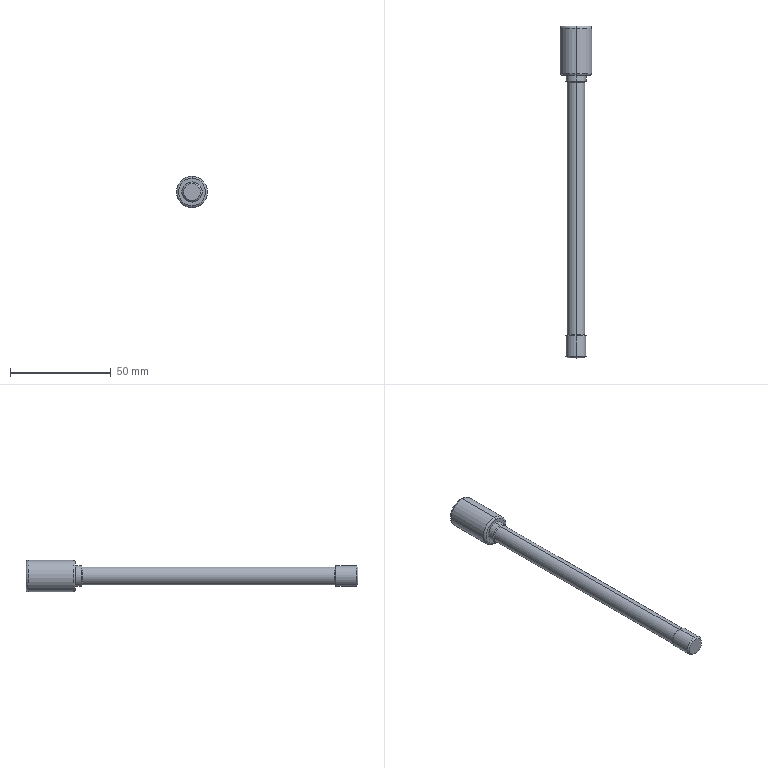Component | SolidWorks | AirTACCylinderFSC_80x75_S_FB-1_FSC80_753-1 | 1 solid | 38 faces | box 15.5 x 164.5 x 15.5 mm | volume 12478 mm3 | plane 16 | cylinder 10 | cone 8 | torus 4 | commonest cylinder face diameters 10 x4 8.9 x2 15.5 x2 8.376 x2
build123d program:
from build123d import *

# Parameters (mm, degrees)
CUT_EXTRUDE1_DEPTH = 4.5


with BuildPart() as part:
    # Sketch1 → Revolve1 (revolve)
    with BuildSketch(Plane.XY, mode=Mode.PRIVATE) as revolve1_sk:
        with BuildLine():
            Line((-24.5, 0), (-24.5, 6.75))
            ThreePointArc((-24.5, 6.75), (-24.207, 7.457), (-23.5, 7.75))
            Line((-23.5, 7.75), (-1, 7.75))
            ThreePointArc((-1, 7.75), (-0.2929, 7.457), (0, 6.75))
            Line((0, 6.75), (0, 0))
            Line((0, 0), (-24.5, 0))
        make_face()
    revolve(revolve1_sk.sketch.rotate(Axis((0, 0, 0), (-1, 0, 0)), 270), axis=Axis((0, 0, 0), (-1, 0, 0)))

    # Sketch2 → Cut-Extrude1 (cut)
    with BuildSketch(Plane(origin=(-24.5, 0, 0), x_dir=(0, 0, -1), z_dir=(1, 0, 0))):
        Polygon((-5, 2.887), (-5, -2.887), (0, -5.774), (5, -2.887), (5, 2.887), (0, 5.774), align=None)
    extrude(amount=CUT_EXTRUDE1_DEPTH, mode=Mode.SUBTRACT)

    # Sketch3 → Cut-Revolve1 (revolve, cut)
    with BuildSketch(Plane.XY, mode=Mode.PRIVATE) as cut_revolve1_sk:
        Polygon((-20, 0), (-20, 5), (-19.188, 4.188), (-0.812, 4.188), (0, 5), (0, 0), align=None)
    revolve(cut_revolve1_sk.sketch.rotate(Axis((0, 0, 0), (-1, 0, 0)), 270), axis=Axis((0, 0, 0), (-1, 0, 0)), mode=Mode.SUBTRACT)

    # Sketch4 → Revolve2 (revolve)
    with BuildSketch(Plane.XY, mode=Mode.PRIVATE) as revolve2_sk:
        Polygon((-8, 0), (-8, 4.2), (-7.2, 5), (2.95, 5), (3.5, 4.45), (128.5, 4.45), (129.05, 5), (139.2, 5), (140, 4.2), (140, 0), align=None)
    revolve(revolve2_sk.sketch.rotate(Axis((140, 0, 0), (-1, 0, 0)), 270), axis=Axis((140, 0, 0), (-1, 0, 0)))


solid = part.part

# Placed as in the assembly
solid = solid.moved(Location((-35, 173, 35), (0, 0, -90)))
STEP:
#1=COLOUR_RGB('',0.7922,0.8196,0.9333);
#2=FILL_AREA_STYLE_COLOUR('',#1);
#3=FILL_AREA_STYLE('',(#2));
#4=SURFACE_STYLE_FILL_AREA(#3);
#5=SURFACE_SIDE_STYLE('',(#4));
#6=SURFACE_STYLE_USAGE(.BOTH.,#5);
#7=PRESENTATION_STYLE_ASSIGNMENT((#6));
#8=CARTESIAN_POINT('',(-1.378,6.695,1.575));
#9=VERTEX_POINT('',#8);
#10=CARTESIAN_POINT('',(-1.378,6.695,1.181));
#11=VERTEX_POINT('',#10);
#12=CARTESIAN_POINT('',(-1.378,6.695,1.378));
#13=DIRECTION('',(0.,1.,0.));
#14=DIRECTION('',(0.,0.,1.));
#15=AXIS2_PLACEMENT_3D('',#12,#13,#14);
#16=CIRCLE('',#15,0.1969);
#17=EDGE_CURVE('',#9,#11,#16,.T.);
#18=ORIENTED_EDGE('',*,*,#17,.T.);
#19=CARTESIAN_POINT('',(-1.378,6.811,1.181));
#20=VERTEX_POINT('',#19);
#21=CARTESIAN_POINT('',(-1.378,1.299,1.181));
#22=DIRECTION('',(0.,1.,0.));
#23=VECTOR('',#22,39.37);
#24=LINE('',#21,#23);
#25=EDGE_CURVE('',#11,#20,#24,.T.);
#26=ORIENTED_EDGE('',*,*,#25,.T.);
#27=CARTESIAN_POINT('',(-1.378,6.811,1.575));
#28=VERTEX_POINT('',#27);
#29=CARTESIAN_POINT('',(-1.378,6.811,1.378));
#30=DIRECTION('',(0.,1.,0.));
#31=DIRECTION('',(0.,0.,-1.));
#32=AXIS2_PLACEMENT_3D('',#29,#30,#31);
#33=CIRCLE('',#32,0.1969);
#34=EDGE_CURVE('',#28,#20,#33,.T.);
#35=ORIENTED_EDGE('',*,*,#34,.F.);
#36=CARTESIAN_POINT('',(-1.378,1.299,1.575));
#37=DIRECTION('',(0.,1.,0.));
#38=VECTOR('',#37,39.37);
#39=LINE('',#36,#38);
#40=EDGE_CURVE('',#9,#28,#39,.T.);
#41=ORIENTED_EDGE('',*,*,#40,.F.);
#42=EDGE_LOOP('',(#18,#26,#35,#41));
#43=FACE_OUTER_BOUND('',#42,.T.);
#44=CARTESIAN_POINT('',(-1.378,1.299,1.378));
#45=DIRECTION('',(0.,1.,0.));
#46=DIRECTION('',(0.,0.,1.));
#47=AXIS2_PLACEMENT_3D('',#44,#45,#46);
#48=CYLINDRICAL_SURFACE('',#47,0.1969);
#49=ADVANCED_FACE('',(#43),#48,.T.);
#50=CARTESIAN_POINT('',(-1.378,6.673,1.553));
#51=VERTEX_POINT('',#50);
#52=CARTESIAN_POINT('',(-1.378,6.673,1.203));
#53=VERTEX_POINT('',#52);
#54=CARTESIAN_POINT('',(-1.378,6.673,1.378));
#55=DIRECTION('',(0.,1.,0.));
#56=DIRECTION('',(0.,0.,1.));
#57=AXIS2_PLACEMENT_3D('',#54,#55,#56);
#58=CIRCLE('',#57,0.1752);
#59=EDGE_CURVE('',#51,#53,#58,.T.);
#60=ORIENTED_EDGE('',*,*,#59,.T.);
#61=CARTESIAN_POINT('',(-1.378,6.673,1.203));
#62=DIRECTION('',(0.,0.7071,-0.7071));
#63=VECTOR('',#62,39.37);
#64=LINE('',#61,#63);
#65=EDGE_CURVE('',#53,#11,#64,.T.);
#66=ORIENTED_EDGE('',*,*,#65,.T.);
#67=ORIENTED_EDGE('',*,*,#17,.F.);
#68=CARTESIAN_POINT('',(-1.378,6.673,1.553));
#69=DIRECTION('',(0.,0.7071,0.7071));
#70=VECTOR('',#69,39.37);
#71=LINE('',#68,#70);
#72=EDGE_CURVE('',#51,#9,#71,.T.);
#73=ORIENTED_EDGE('',*,*,#72,.F.);
#74=EDGE_LOOP('',(#60,#66,#67,#73));
#75=FACE_OUTER_BOUND('',#74,.T.);
#76=CARTESIAN_POINT('',(-1.378,6.673,1.378));
#77=DIRECTION('',(0.,1.,0.));
#78=DIRECTION('',(0.,0.,1.));
#79=AXIS2_PLACEMENT_3D('',#76,#77,#78);
#80=CONICAL_SURFACE('',#79,0.1752,0.7854);
#81=ADVANCED_FACE('',(#75),#80,.T.);
#82=CARTESIAN_POINT('',(-1.378,1.752,1.553));
#83=VERTEX_POINT('',#82);
#84=CARTESIAN_POINT('',(-1.378,1.752,1.203));
#85=VERTEX_POINT('',#84);
#86=CARTESIAN_POINT('',(-1.378,1.752,1.378));
#87=DIRECTION('',(0.,1.,0.));
#88=DIRECTION('',(0.,0.,1.));
#89=AXIS2_PLACEMENT_3D('',#86,#87,#88);
#90=CIRCLE('',#89,0.1752);
#91=EDGE_CURVE('',#83,#85,#90,.T.);
#92=ORIENTED_EDGE('',*,*,#91,.T.);
#93=CARTESIAN_POINT('',(-1.378,1.299,1.203));
#94=DIRECTION('',(0.,1.,0.));
#95=VECTOR('',#94,39.37);
#96=LINE('',#93,#95);
#97=EDGE_CURVE('',#85,#53,#96,.T.);
#98=ORIENTED_EDGE('',*,*,#97,.T.);
#99=ORIENTED_EDGE('',*,*,#59,.F.);
#100=CARTESIAN_POINT('',(-1.378,1.299,1.553));
#101=DIRECTION('',(0.,1.,0.));
#102=VECTOR('',#101,39.37);
#103=LINE('',#100,#102);
#104=EDGE_CURVE('',#83,#51,#103,.T.);
#105=ORIENTED_EDGE('',*,*,#104,.F.);
#106=EDGE_LOOP('',(#92,#98,#99,#105));
#107=FACE_OUTER_BOUND('',#106,.T.);
#108=CARTESIAN_POINT('',(-1.378,1.299,1.378));
#109=DIRECTION('',(0.,1.,0.));
#110=DIRECTION('',(0.,0.,1.));
#111=AXIS2_PLACEMENT_3D('',#108,#109,#110);
#112=CYLINDRICAL_SURFACE('',#111,0.1752);
#113=ADVANCED_FACE('',(#107),#112,.T.);
#114=ORIENTED_EDGE('',*,*,#91,.F.);
#115=CARTESIAN_POINT('',(-1.378,1.73,1.575));
#116=VERTEX_POINT('',#115);
#117=CARTESIAN_POINT('',(-1.378,1.73,1.575));
#118=DIRECTION('',(0.,-0.7071,0.7071));
#119=VECTOR('',#118,39.37);
#120=LINE('',#117,#119);
#121=EDGE_CURVE('',#83,#116,#120,.T.);
#122=ORIENTED_EDGE('',*,*,#121,.T.);
#123=CARTESIAN_POINT('',(-1.378,1.73,1.181));
#124=VERTEX_POINT('',#123);
#125=CARTESIAN_POINT('',(-1.378,1.73,1.378));
#126=DIRECTION('',(0.,1.,0.));
#127=DIRECTION('',(0.,0.,1.));
#128=AXIS2_PLACEMENT_3D('',#125,#126,#127);
#129=CIRCLE('',#128,0.1969);
#130=EDGE_CURVE('',#116,#124,#129,.T.);
#131=ORIENTED_EDGE('',*,*,#130,.T.);
#132=CARTESIAN_POINT('',(-1.378,1.73,1.181));
#133=DIRECTION('',(0.,-0.7071,-0.7071));
#134=VECTOR('',#133,39.37);
#135=LINE('',#132,#134);
#136=EDGE_CURVE('',#85,#124,#135,.T.);
#137=ORIENTED_EDGE('',*,*,#136,.F.);
#138=EDGE_LOOP('',(#114,#122,#131,#137));
#139=FACE_OUTER_BOUND('',#138,.T.);
#140=CARTESIAN_POINT('',(-1.378,1.73,1.378));
#141=DIRECTION('',(0.,-1.,0.));
#142=DIRECTION('',(0.,0.,-1.));
#143=AXIS2_PLACEMENT_3D('',#140,#141,#142);
#144=CONICAL_SURFACE('',#143,0.1969,0.7854);
#145=ADVANCED_FACE('',(#139),#144,.T.);
#146=CARTESIAN_POINT('',(-1.378,1.331,1.575));
#147=VERTEX_POINT('',#146);
#148=CARTESIAN_POINT('',(-1.378,1.331,1.181));
#149=VERTEX_POINT('',#148);
#150=CARTESIAN_POINT('',(-1.378,1.331,1.378));
#151=DIRECTION('',(0.,1.,0.));
#152=DIRECTION('',(0.,0.,1.));
#153=AXIS2_PLACEMENT_3D('',#150,#151,#152);
#154=CIRCLE('',#153,0.1969);
#155=EDGE_CURVE('',#147,#149,#154,.T.);
#156=ORIENTED_EDGE('',*,*,#155,.T.);
#157=CARTESIAN_POINT('',(-1.378,1.299,1.181));
#158=DIRECTION('',(0.,1.,0.));
#159=VECTOR('',#158,39.37);
#160=LINE('',#157,#159);
#161=EDGE_CURVE('',#149,#124,#160,.T.);
#162=ORIENTED_EDGE('',*,*,#161,.T.);
#163=ORIENTED_EDGE('',*,*,#130,.F.);
#164=CARTESIAN_POINT('',(-1.378,1.299,1.575));
#165=DIRECTION('',(0.,1.,0.));
#166=VECTOR('',#165,39.37);
#167=LINE('',#164,#166);
#168=EDGE_CURVE('',#147,#116,#167,.T.);
#169=ORIENTED_EDGE('',*,*,#168,.F.);
#170=EDGE_LOOP('',(#156,#162,#163,#169));
#171=FACE_OUTER_BOUND('',#170,.T.);
#172=CARTESIAN_POINT('',(-1.378,1.299,1.378));
#173=DIRECTION('',(0.,1.,0.));
#174=DIRECTION('',(0.,0.,1.));
#175=AXIS2_PLACEMENT_3D('',#172,#173,#174);
#176=CYLINDRICAL_SURFACE('',#175,0.1969);
#177=ADVANCED_FACE('',(#171),#176,.T.);
#178=CARTESIAN_POINT('',(-1.378,1.299,1.543));
#179=VERTEX_POINT('',#178);
#180=CARTESIAN_POINT('',(-1.378,1.299,1.213));
#181=VERTEX_POINT('',#180);
#182=CARTESIAN_POINT('',(-1.378,1.299,1.378));
#183=DIRECTION('',(0.,1.,0.));
#184=DIRECTION('',(0.,0.,1.));
#185=AXIS2_PLACEMENT_3D('',#182,#183,#184);
#186=CIRCLE('',#185,0.1654);
#187=EDGE_CURVE('',#179,#181,#186,.T.);
#188=ORIENTED_EDGE('',*,*,#187,.T.);
#189=CARTESIAN_POINT('',(-1.378,1.299,1.213));
#190=DIRECTION('',(0.,0.7071,-0.7071));
#191=VECTOR('',#190,39.37);
#192=LINE('',#189,#191);
#193=EDGE_CURVE('',#181,#149,#192,.T.);
#194=ORIENTED_EDGE('',*,*,#193,.T.);
#195=ORIENTED_EDGE('',*,*,#155,.F.);
#196=CARTESIAN_POINT('',(-1.378,1.299,1.543));
#197=DIRECTION('',(0.,0.7071,0.7071));
#198=VECTOR('',#197,39.37);
#199=LINE('',#196,#198);
#200=EDGE_CURVE('',#179,#147,#199,.T.);
#201=ORIENTED_EDGE('',*,*,#200,.F.);
#202=EDGE_LOOP('',(#188,#194,#195,#201));
#203=FACE_OUTER_BOUND('',#202,.T.);
#204=CARTESIAN_POINT('',(-1.378,1.299,1.378));
#205=DIRECTION('',(0.,1.,0.));
#206=DIRECTION('',(0.,0.,1.));
#207=AXIS2_PLACEMENT_3D('',#204,#205,#206);
#208=CONICAL_SURFACE('',#207,0.1654,0.7854);
#209=ADVANCED_FACE('',(#203),#208,.T.);
#210=CARTESIAN_POINT('',(-1.378,7.566,1.213));
#211=VERTEX_POINT('',#210);
#212=CARTESIAN_POINT('',(-1.378,7.566,1.543));
#213=VERTEX_POINT('',#212);
#214=CARTESIAN_POINT('',(-1.378,7.566,1.378));
#215=DIRECTION('',(0.,1.,0.));
#216=DIRECTION('',(0.,0.,1.));
#217=AXIS2_PLACEMENT_3D('',#214,#215,#216);
#218=CIRCLE('',#217,0.1649);
#219=EDGE_CURVE('',#211,#213,#218,.T.);
#220=ORIENTED_EDGE('',*,*,#219,.F.);
#221=CARTESIAN_POINT('',(-1.378,7.598,1.181));
#222=VERTEX_POINT('',#221);
#223=CARTESIAN_POINT('',(-1.378,7.566,1.213));
#224=DIRECTION('',(0.,0.7071,-0.7071));
#225=VECTOR('',#224,39.37);
#226=LINE('',#223,#225);
#227=EDGE_CURVE('',#211,#222,#226,.T.);
#228=ORIENTED_EDGE('',*,*,#227,.T.);
#229=CARTESIAN_POINT('',(-1.548,7.598,1.28));
#230=VERTEX_POINT('',#229);
#231=CARTESIAN_POINT('',(-1.378,7.598,1.378));
#232=DIRECTION('',(0.,1.,0.));
#233=DIRECTION('',(0.,0.,1.));
#234=AXIS2_PLACEMENT_3D('',#231,#232,#233);
#235=CIRCLE('',#234,0.1969);
#236=EDGE_CURVE('',#222,#230,#235,.T.);
#237=ORIENTED_EDGE('',*,*,#236,.T.);
#238=CARTESIAN_POINT('',(-1.548,7.598,1.476));
#239=VERTEX_POINT('',#238);
#240=CARTESIAN_POINT('',(-1.378,7.598,1.378));
#241=DIRECTION('',(0.,1.,0.));
#242=DIRECTION('',(0.,0.,1.));
#243=AXIS2_PLACEMENT_3D('',#240,#241,#242);
#244=CIRCLE('',#243,0.1969);
#245=EDGE_CURVE('',#230,#239,#244,.T.);
#246=ORIENTED_EDGE('',*,*,#245,.T.);
#247=CARTESIAN_POINT('',(-1.378,7.598,1.575));
#248=VERTEX_POINT('',#247);
#249=CARTESIAN_POINT('',(-1.378,7.598,1.378));
#250=DIRECTION('',(0.,1.,0.));
#251=DIRECTION('',(0.,0.,1.));
#252=AXIS2_PLACEMENT_3D('',#249,#250,#251);
#253=CIRCLE('',#252,0.1969);
#254=EDGE_CURVE('',#239,#248,#253,.T.);
#255=ORIENTED_EDGE('',*,*,#254,.T.);
#256=CARTESIAN_POINT('',(-1.378,7.566,1.543));
#257=DIRECTION('',(0.,0.7071,0.7071));
#258=VECTOR('',#257,39.37);
#259=LINE('',#256,#258);
#260=EDGE_CURVE('',#213,#248,#259,.T.);
#261=ORIENTED_EDGE('',*,*,#260,.F.);
#262=EDGE_LOOP('',(#220,#228,#237,#246,#255,#261));
#263=FACE_OUTER_BOUND('',#262,.T.);
#264=CARTESIAN_POINT('',(-1.378,7.566,1.378));
#265=DIRECTION('',(0.,1.,0.));
#266=DIRECTION('',(0.,0.,1.));
#267=AXIS2_PLACEMENT_3D('',#264,#265,#266);
#268=CONICAL_SURFACE('',#267,0.1649,0.7854);
#269=ADVANCED_FACE('',(#263),#268,.F.);
#270=CARTESIAN_POINT('',(-1.378,6.811,1.644));
#271=VERTEX_POINT('',#270);
#272=CARTESIAN_POINT('',(-1.378,6.811,1.112));
#273=VERTEX_POINT('',#272);
#274=CARTESIAN_POINT('',(-1.378,6.811,1.378));
#275=DIRECTION('',(0.,1.,0.));
#276=DIRECTION('',(0.,0.,1.));
#277=AXIS2_PLACEMENT_3D('',#274,#275,#276);
#278=CIRCLE('',#277,0.2657);
#279=EDGE_CURVE('',#271,#273,#278,.T.);
#280=ORIENTED_EDGE('',*,*,#279,.T.);
#281=CARTESIAN_POINT('',(-1.378,6.85,1.073));
#282=VERTEX_POINT('',#281);
#283=CARTESIAN_POINT('',(-1.378,6.85,1.112));
#284=DIRECTION('',(1.,0.,0.));
#285=DIRECTION('',(0.,0.,-1.));
#286=AXIS2_PLACEMENT_3D('',#283,#284,#285);
#287=CIRCLE('',#286,0.03937);
#288=EDGE_CURVE('',#273,#282,#287,.T.);
#289=ORIENTED_EDGE('',*,*,#288,.T.);
#290=CARTESIAN_POINT('',(-1.378,6.85,1.683));
#291=VERTEX_POINT('',#290);
#292=CARTESIAN_POINT('',(-1.378,6.85,1.378));
#293=DIRECTION('',(0.,1.,0.));
#294=DIRECTION('',(0.,0.,1.));
#295=AXIS2_PLACEMENT_3D('',#292,#293,#294);
#296=CIRCLE('',#295,0.3051);
#297=EDGE_CURVE('',#291,#282,#296,.T.);
#298=ORIENTED_EDGE('',*,*,#297,.F.);
#299=CARTESIAN_POINT('',(-1.378,6.85,1.644));
#300=DIRECTION('',(-1.,0.,0.));
#301=DIRECTION('',(0.,0.,1.));
#302=AXIS2_PLACEMENT_3D('',#299,#300,#301);
#303=CIRCLE('',#302,0.03937);
#304=EDGE_CURVE('',#271,#291,#303,.T.);
#305=ORIENTED_EDGE('',*,*,#304,.F.);
#306=EDGE_LOOP('',(#280,#289,#298,#305));
#307=FACE_OUTER_BOUND('',#306,.T.);
#308=CARTESIAN_POINT('',(-1.378,6.85,1.378));
#309=DIRECTION('',(0.,1.,0.));
#310=DIRECTION('',(0.,0.,1.));
#311=AXIS2_PLACEMENT_3D('',#308,#309,#310);
#312=TOROIDAL_SURFACE('',#311,0.2657,0.03937);
#313=ADVANCED_FACE('',(#307),#312,.T.);
#314=ORIENTED_EDGE('',*,*,#297,.T.);
#315=CARTESIAN_POINT('',(-1.378,7.736,1.073));
#316=VERTEX_POINT('',#315);
#317=CARTESIAN_POINT('',(-1.378,6.811,1.073));
#318=DIRECTION('',(0.,1.,0.));
#319=VECTOR('',#318,39.37);
#320=LINE('',#317,#319);
#321=EDGE_CURVE('',#282,#316,#320,.T.);
#322=ORIENTED_EDGE('',*,*,#321,.T.);
#323=CARTESIAN_POINT('',(-1.378,7.736,1.683));
#324=VERTEX_POINT('',#323);
#325=CARTESIAN_POINT('',(-1.378,7.736,1.378));
#326=DIRECTION('',(0.,1.,0.));
#327=DIRECTION('',(0.,0.,1.));
#328=AXIS2_PLACEMENT_3D('',#325,#326,#327);
#329=CIRCLE('',#328,0.3051);
#330=EDGE_CURVE('',#324,#316,#329,.T.);
#331=ORIENTED_EDGE('',*,*,#330,.F.);
#332=CARTESIAN_POINT('',(-1.378,6.811,1.683));
#333=DIRECTION('',(0.,1.,0.));
#334=VECTOR('',#333,39.37);
#335=LINE('',#332,#334);
#336=EDGE_CURVE('',#291,#324,#335,.T.);
#337=ORIENTED_EDGE('',*,*,#336,.F.);
#338=EDGE_LOOP('',(#314,#322,#331,#337));
#339=FACE_OUTER_BOUND('',#338,.T.);
#340=CARTESIAN_POINT('',(-1.378,6.811,1.378));
#341=DIRECTION('',(0.,1.,0.));
#342=DIRECTION('',(0.,0.,1.));
#343=AXIS2_PLACEMENT_3D('',#340,#341,#342);
#344=CYLINDRICAL_SURFACE('',#343,0.3051);
#345=ADVANCED_FACE('',(#339),#344,.T.);
#346=ORIENTED_EDGE('',*,*,#330,.T.);
#347=CARTESIAN_POINT('',(-1.378,7.776,1.112));
#348=VERTEX_POINT('',#347);
#349=CARTESIAN_POINT('',(-1.378,7.736,1.112));
#350=DIRECTION('',(1.,0.,0.));
#351=DIRECTION('',(0.,0.,-1.));
#352=AXIS2_PLACEMENT_3D('',#349,#350,#351);
#353=CIRCLE('',#352,0.03937);
#354=EDGE_CURVE('',#316,#348,#353,.T.);
#355=ORIENTED_EDGE('',*,*,#354,.T.);
#356=CARTESIAN_POINT('',(-1.378,7.776,1.644));
#357=VERTEX_POINT('',#356);
#358=CARTESIAN_POINT('',(-1.378,7.776,1.378));
#359=DIRECTION('',(0.,1.,0.));
#360=DIRECTION('',(0.,0.,1.));
#361=AXIS2_PLACEMENT_3D('',#358,#359,#360);
#362=CIRCLE('',#361,0.2657);
#363=EDGE_CURVE('',#357,#348,#362,.T.);
#364=ORIENTED_EDGE('',*,*,#363,.F.);
#365=CARTESIAN_POINT('',(-1.378,7.736,1.644));
#366=DIRECTION('',(-1.,0.,0.));
#367=DIRECTION('',(0.,0.,1.));
#368=AXIS2_PLACEMENT_3D('',#365,#366,#367);
#369=CIRCLE('',#368,0.03937);
#370=EDGE_CURVE('',#324,#357,#369,.T.);
#371=ORIENTED_EDGE('',*,*,#370,.F.);
#372=EDGE_LOOP('',(#346,#355,#364,#371));
#373=FACE_OUTER_BOUND('',#372,.T.);
#374=CARTESIAN_POINT('',(-1.378,7.736,1.378));
#375=DIRECTION('',(0.,1.,0.));
#376=DIRECTION('',(0.,0.,1.));
#377=AXIS2_PLACEMENT_3D('',#374,#375,#376);
#378=TOROIDAL_SURFACE('',#377,0.2657,0.03937);
#379=ADVANCED_FACE('',(#373),#378,.T.);
#380=CARTESIAN_POINT('',(-1.378,7.126,1.543));
#381=VERTEX_POINT('',#380);
#382=CARTESIAN_POINT('',(-1.378,7.126,1.213));
#383=VERTEX_POINT('',#382);
#384=CARTESIAN_POINT('',(-1.378,7.126,1.378));
#385=DIRECTION('',(0.,-1.,0.));
#386=DIRECTION('',(0.,0.,-1.));
#387=AXIS2_PLACEMENT_3D('',#384,#385,#386);
#388=CIRCLE('',#387,0.1649);
#389=EDGE_CURVE('',#381,#383,#388,.T.);
#390=ORIENTED_EDGE('',*,*,#389,.T.);
#391=CARTESIAN_POINT('',(-1.378,6.811,1.213));
#392=DIRECTION('',(0.,1.,0.));
#393=VECTOR('',#392,39.37);
#394=LINE('',#391,#393);
#395=EDGE_CURVE('',#383,#211,#394,.T.);
#396=ORIENTED_EDGE('',*,*,#395,.T.);
#397=ORIENTED_EDGE('',*,*,#219,.T.);
#398=CARTESIAN_POINT('',(-1.378,6.811,1.543));
#399=DIRECTION('',(0.,1.,0.));
#400=VECTOR('',#399,39.37);
#401=LINE('',#398,#400);
#402=EDGE_CURVE('',#381,#213,#401,.T.);
#403=ORIENTED_EDGE('',*,*,#402,.F.);
#404=EDGE_LOOP('',(#390,#396,#397,#403));
#405=FACE_OUTER_BOUND('',#404,.T.);
#406=CARTESIAN_POINT('',(-1.378,6.811,1.378));
#407=DIRECTION('',(0.,1.,0.));
#408=DIRECTION('',(0.,0.,1.));
#409=AXIS2_PLACEMENT_3D('',#406,#407,#408);
#410=CYLINDRICAL_SURFACE('',#409,0.1649);
#411=ADVANCED_FACE('',(#405),#410,.F.);
#412=ORIENTED_EDGE('',*,*,#395,.F.);
#413=CARTESIAN_POINT('',(-1.378,7.126,1.378));
#414=DIRECTION('',(0.,-1.,0.));
#415=DIRECTION('',(0.,0.,-1.));
#416=AXIS2_PLACEMENT_3D('',#413,#414,#415);
#417=CIRCLE('',#416,0.1649);
#418=EDGE_CURVE('',#383,#381,#417,.T.);
#419=ORIENTED_EDGE('',*,*,#418,.T.);
#420=ORIENTED_EDGE('',*,*,#402,.T.);
#421=CARTESIAN_POINT('',(-1.378,7.566,1.378));
#422=DIRECTION('',(0.,1.,0.));
#423=DIRECTION('',(0.,0.,1.));
#424=AXIS2_PLACEMENT_3D('',#421,#422,#423);
#425=CIRCLE('',#424,0.1649);
#426=EDGE_CURVE('',#213,#211,#425,.T.);
#427=ORIENTED_EDGE('',*,*,#426,.T.);
#428=EDGE_LOOP('',(#412,#419,#420,#427));
#429=FACE_OUTER_BOUND('',#428,.T.);
#430=CARTESIAN_POINT('',(-1.378,6.811,1.378));
#431=DIRECTION('',(0.,1.,0.));
#432=DIRECTION('',(0.,0.,1.));
#433=AXIS2_PLACEMENT_3D('',#430,#431,#432);
#434=CYLINDRICAL_SURFACE('',#433,0.1649);
#435=ADVANCED_FACE('',(#429),#434,.F.);
#436=CARTESIAN_POINT('',(-1.207,7.598,1.476));
#437=VERTEX_POINT('',#436);
#438=CARTESIAN_POINT('',(-1.378,7.598,1.378));
#439=DIRECTION('',(0.,1.,0.));
#440=DIRECTION('',(0.,0.,1.));
#441=AXIS2_PLACEMENT_3D('',#438,#439,#440);
#442=CIRCLE('',#441,0.1969);
#443=EDGE_CURVE('',#248,#437,#442,.T.);
#444=ORIENTED_EDGE('',*,*,#443,.F.);
#445=CARTESIAN_POINT('',(-1.264,7.598,1.575));
#446=VERTEX_POINT('',#445);
#447=CARTESIAN_POINT('',(-1.264,7.598,1.575));
#448=DIRECTION('',(-1.,0.,0.));
#449=VECTOR('',#448,39.37);
#450=LINE('',#447,#449);
#451=EDGE_CURVE('',#446,#248,#450,.T.);
#452=ORIENTED_EDGE('',*,*,#451,.F.);
#453=CARTESIAN_POINT('',(-1.151,7.598,1.378));
#454=DIRECTION('',(-0.5,0.,0.866));
#455=VECTOR('',#454,39.37);
#456=LINE('',#453,#455);
#457=EDGE_CURVE('',#437,#446,#456,.T.);
#458=ORIENTED_EDGE('',*,*,#457,.F.);
#459=EDGE_LOOP('',(#444,#452,#458));
#460=FACE_OUTER_BOUND('',#459,.T.);
#461=CARTESIAN_POINT('',(-1.264,7.598,1.575));
#462=DIRECTION('',(0.,-1.,0.));
#463=DIRECTION('',(0.,0.,-1.));
#464=AXIS2_PLACEMENT_3D('',#461,#462,#463);
#465=PLANE('',#464);
#466=ADVANCED_FACE('',(#460),#465,.F.);
#467=CARTESIAN_POINT('',(-1.207,7.598,1.28));
#468=VERTEX_POINT('',#467);
#469=CARTESIAN_POINT('',(-1.378,7.598,1.378));
#470=DIRECTION('',(0.,1.,0.));
#471=DIRECTION('',(0.,0.,1.));
#472=AXIS2_PLACEMENT_3D('',#469,#470,#471);
#473=CIRCLE('',#472,0.1969);
#474=EDGE_CURVE('',#437,#468,#473,.T.);
#475=ORIENTED_EDGE('',*,*,#474,.F.);
#476=CARTESIAN_POINT('',(-1.151,7.598,1.378));
#477=VERTEX_POINT('',#476);
#478=CARTESIAN_POINT('',(-1.151,7.598,1.378));
#479=DIRECTION('',(-0.5,0.,0.866));
#480=VECTOR('',#479,39.37);
#481=LINE('',#478,#480);
#482=EDGE_CURVE('',#477,#437,#481,.T.);
#483=ORIENTED_EDGE('',*,*,#482,.F.);
#484=CARTESIAN_POINT('',(-1.264,7.598,1.181));
#485=DIRECTION('',(0.5,0.,0.866));
#486=VECTOR('',#485,39.37);
#487=LINE('',#484,#486);
#488=EDGE_CURVE('',#468,#477,#487,.T.);
#489=ORIENTED_EDGE('',*,*,#488,.F.);
#490=EDGE_LOOP('',(#475,#483,#489));
#491=FACE_OUTER_BOUND('',#490,.T.);
#492=CARTESIAN_POINT('',(-1.264,7.598,1.575));
#493=DIRECTION('',(0.,-1.,0.));
#494=DIRECTION('',(0.,0.,-1.));
#495=AXIS2_PLACEMENT_3D('',#492,#493,#494);
#496=PLANE('',#495);
#497=ADVANCED_FACE('',(#491),#496,.F.);
#498=CARTESIAN_POINT('',(-1.378,7.598,1.378));
#499=DIRECTION('',(0.,1.,0.));
#500=DIRECTION('',(0.,0.,1.));
#501=AXIS2_PLACEMENT_3D('',#498,#499,#500);
#502=CIRCLE('',#501,0.1969);
#503=EDGE_CURVE('',#468,#222,#502,.T.);
#504=ORIENTED_EDGE('',*,*,#503,.F.);
#505=CARTESIAN_POINT('',(-1.264,7.598,1.181));
#506=VERTEX_POINT('',#505);
#507=CARTESIAN_POINT('',(-1.264,7.598,1.181));
#508=DIRECTION('',(0.5,0.,0.866));
#509=VECTOR('',#508,39.37);
#510=LINE('',#507,#509);
#511=EDGE_CURVE('',#506,#468,#510,.T.);
#512=ORIENTED_EDGE('',*,*,#511,.F.);
#513=CARTESIAN_POINT('',(-1.492,7.598,1.181));
#514=DIRECTION('',(1.,0.,0.));
#515=VECTOR('',#514,39.37);
#516=LINE('',#513,#515);
#517=EDGE_CURVE('',#222,#506,#516,.T.);
#518=ORIENTED_EDGE('',*,*,#517,.F.);
#519=EDGE_LOOP('',(#504,#512,#518));
#520=FACE_OUTER_BOUND('',#519,.T.);
#521=CARTESIAN_POINT('',(-1.264,7.598,1.575));
#522=DIRECTION('',(0.,-1.,0.));
#523=DIRECTION('',(0.,0.,-1.));
#524=AXIS2_PLACEMENT_3D('',#521,#522,#523);
#525=PLANE('',#524);
#526=ADVANCED_FACE('',(#520),#525,.F.);
#527=ORIENTED_EDGE('',*,*,#236,.F.);
#528=CARTESIAN_POINT('',(-1.492,7.598,1.181));
#529=VERTEX_POINT('',#528);
#530=CARTESIAN_POINT('',(-1.492,7.598,1.181));
#531=DIRECTION('',(1.,0.,0.));
#532=VECTOR('',#531,39.37);
#533=LINE('',#530,#532);
#534=EDGE_CURVE('',#529,#222,#533,.T.);
#535=ORIENTED_EDGE('',*,*,#534,.F.);
#536=CARTESIAN_POINT('',(-1.605,7.598,1.378));
#537=DIRECTION('',(0.5,0.,-0.866));
#538=VECTOR('',#537,39.37);
#539=LINE('',#536,#538);
#540=EDGE_CURVE('',#230,#529,#539,.T.);
#541=ORIENTED_EDGE('',*,*,#540,.F.);
#542=EDGE_LOOP('',(#527,#535,#541));
#543=FACE_OUTER_BOUND('',#542,.T.);
#544=CARTESIAN_POINT('',(-1.264,7.598,1.575));
#545=DIRECTION('',(0.,-1.,0.));
#546=DIRECTION('',(0.,0.,-1.));
#547=AXIS2_PLACEMENT_3D('',#544,#545,#546);
#548=PLANE('',#547);
#549=ADVANCED_FACE('',(#543),#548,.F.);
#550=ORIENTED_EDGE('',*,*,#245,.F.);
#551=CARTESIAN_POINT('',(-1.605,7.598,1.378));
#552=VERTEX_POINT('',#551);
#553=CARTESIAN_POINT('',(-1.605,7.598,1.378));
#554=DIRECTION('',(0.5,0.,-0.866));
#555=VECTOR('',#554,39.37);
#556=LINE('',#553,#555);
#557=EDGE_CURVE('',#552,#230,#556,.T.);
#558=ORIENTED_EDGE('',*,*,#557,.F.);
#559=CARTESIAN_POINT('',(-1.492,7.598,1.575));
#560=DIRECTION('',(-0.5,0.,-0.866));
#561=VECTOR('',#560,39.37);
#562=LINE('',#559,#561);
#563=EDGE_CURVE('',#239,#552,#562,.T.);
#564=ORIENTED_EDGE('',*,*,#563,.F.);
#565=EDGE_LOOP('',(#550,#558,#564));
#566=FACE_OUTER_BOUND('',#565,.T.);
#567=CARTESIAN_POINT('',(-1.264,7.598,1.575));
#568=DIRECTION('',(0.,-1.,0.));
#569=DIRECTION('',(0.,0.,-1.));
#570=AXIS2_PLACEMENT_3D('',#567,#568,#569);
#571=PLANE('',#570);
#572=ADVANCED_FACE('',(#566),#571,.F.);
#573=ORIENTED_EDGE('',*,*,#254,.F.);
#574=CARTESIAN_POINT('',(-1.492,7.598,1.575));
#575=VERTEX_POINT('',#574);
#576=CARTESIAN_POINT('',(-1.492,7.598,1.575));
#577=DIRECTION('',(-0.5,0.,-0.866));
#578=VECTOR('',#577,39.37);
#579=LINE('',#576,#578);
#580=EDGE_CURVE('',#575,#239,#579,.T.);
#581=ORIENTED_EDGE('',*,*,#580,.F.);
#582=CARTESIAN_POINT('',(-1.264,7.598,1.575));
#583=DIRECTION('',(-1.,0.,0.));
#584=VECTOR('',#583,39.37);
#585=LINE('',#582,#584);
#586=EDGE_CURVE('',#248,#575,#585,.T.);
#587=ORIENTED_EDGE('',*,*,#586,.F.);
#588=EDGE_LOOP('',(#573,#581,#587));
#589=FACE_OUTER_BOUND('',#588,.T.);
#590=CARTESIAN_POINT('',(-1.264,7.598,1.575));
#591=DIRECTION('',(0.,-1.,0.));
#592=DIRECTION('',(0.,0.,-1.));
#593=AXIS2_PLACEMENT_3D('',#590,#591,#592);
#594=PLANE('',#593);
#595=ADVANCED_FACE('',(#589),#594,.F.);
#596=ORIENTED_EDGE('',*,*,#279,.F.);
#597=CARTESIAN_POINT('',(-1.378,6.811,1.378));
#598=DIRECTION('',(0.,1.,0.));
#599=DIRECTION('',(0.,0.,1.));
#600=AXIS2_PLACEMENT_3D('',#597,#598,#599);
#601=CIRCLE('',#600,0.2657);
#602=EDGE_CURVE('',#273,#271,#601,.T.);
#603=ORIENTED_EDGE('',*,*,#602,.F.);
#604=EDGE_LOOP('',(#596,#603));
#605=FACE_OUTER_BOUND('',#604,.T.);
#606=ORIENTED_EDGE('',*,*,#34,.T.);
#607=CARTESIAN_POINT('',(-1.378,6.811,1.378));
#608=DIRECTION('',(0.,1.,0.));
#609=DIRECTION('',(0.,0.,-1.));
#610=AXIS2_PLACEMENT_3D('',#607,#608,#609);
#611=CIRCLE('',#610,0.1969);
#612=EDGE_CURVE('',#20,#28,#611,.T.);
#613=ORIENTED_EDGE('',*,*,#612,.T.);
#614=EDGE_LOOP('',(#606,#613));
#615=FACE_BOUND('',#614,.T.);
#616=CARTESIAN_POINT('',(-1.112,6.811,1.378));
#617=DIRECTION('',(0.,1.,0.));
#618=DIRECTION('',(0.,0.,1.));
#619=AXIS2_PLACEMENT_3D('',#616,#617,#618);
#620=PLANE('',#619);
#621=ADVANCED_FACE('',(#605,#615),#620,.F.);
#622=ORIENTED_EDGE('',*,*,#363,.T.);
#623=CARTESIAN_POINT('',(-1.378,7.776,1.378));
#624=DIRECTION('',(0.,1.,0.));
#625=DIRECTION('',(0.,0.,1.));
#626=AXIS2_PLACEMENT_3D('',#623,#624,#625);
#627=CIRCLE('',#626,0.2657);
#628=EDGE_CURVE('',#348,#357,#627,.T.);
#629=ORIENTED_EDGE('',*,*,#628,.T.);
#630=EDGE_LOOP('',(#622,#629));
#631=FACE_OUTER_BOUND('',#630,.T.);
#632=CARTESIAN_POINT('',(-1.151,7.776,1.378));
#633=VERTEX_POINT('',#632);
#634=CARTESIAN_POINT('',(-1.264,7.776,1.575));
#635=VERTEX_POINT('',#634);
#636=CARTESIAN_POINT('',(-1.151,7.776,1.378));
#637=DIRECTION('',(-0.5,0.,0.866));
#638=VECTOR('',#637,39.37);
#639=LINE('',#636,#638);
#640=EDGE_CURVE('',#633,#635,#639,.T.);
#641=ORIENTED_EDGE('',*,*,#640,.T.);
#642=CARTESIAN_POINT('',(-1.492,7.776,1.575));
#643=VERTEX_POINT('',#642);
#644=CARTESIAN_POINT('',(-1.264,7.776,1.575));
#645=DIRECTION('',(-1.,0.,0.));
#646=VECTOR('',#645,39.37);
#647=LINE('',#644,#646);
#648=EDGE_CURVE('',#635,#643,#647,.T.);
#649=ORIENTED_EDGE('',*,*,#648,.T.);
#650=CARTESIAN_POINT('',(-1.605,7.776,1.378));
#651=VERTEX_POINT('',#650);
#652=CARTESIAN_POINT('',(-1.492,7.776,1.575));
#653=DIRECTION('',(-0.5,0.,-0.866));
#654=VECTOR('',#653,39.37);
#655=LINE('',#652,#654);
#656=EDGE_CURVE('',#643,#651,#655,.T.);
#657=ORIENTED_EDGE('',*,*,#656,.T.);
#658=CARTESIAN_POINT('',(-1.492,7.776,1.181));
#659=VERTEX_POINT('',#658);
#660=CARTESIAN_POINT('',(-1.605,7.776,1.378));
#661=DIRECTION('',(0.5,0.,-0.866));
#662=VECTOR('',#661,39.37);
#663=LINE('',#660,#662);
#664=EDGE_CURVE('',#651,#659,#663,.T.);
#665=ORIENTED_EDGE('',*,*,#664,.T.);
#666=CARTESIAN_POINT('',(-1.264,7.776,1.181));
#667=VERTEX_POINT('',#666);
#668=CARTESIAN_POINT('',(-1.492,7.776,1.181));
#669=DIRECTION('',(1.,0.,0.));
#670=VECTOR('',#669,39.37);
#671=LINE('',#668,#670);
#672=EDGE_CURVE('',#659,#667,#671,.T.);
#673=ORIENTED_EDGE('',*,*,#672,.T.);
#674=CARTESIAN_POINT('',(-1.264,7.776,1.181));
#675=DIRECTION('',(0.5,0.,0.866));
#676=VECTOR('',#675,39.37);
#677=LINE('',#674,#676);
#678=EDGE_CURVE('',#667,#633,#677,.T.);
#679=ORIENTED_EDGE('',*,*,#678,.T.);
#680=EDGE_LOOP('',(#641,#649,#657,#665,#673,#679));
#681=FACE_BOUND('',#680,.T.);
#682=CARTESIAN_POINT('',(-1.378,7.776,1.378));
#683=DIRECTION('',(0.,-1.,0.));
#684=DIRECTION('',(0.,0.,-1.));
#685=AXIS2_PLACEMENT_3D('',#682,#683,#684);
#686=PLANE('',#685);
#687=ADVANCED_FACE('',(#631,#681),#686,.F.);
#688=ORIENTED_EDGE('',*,*,#354,.F.);
#689=CARTESIAN_POINT('',(-1.378,7.736,1.378));
#690=DIRECTION('',(0.,1.,0.));
#691=DIRECTION('',(0.,0.,1.));
#692=AXIS2_PLACEMENT_3D('',#689,#690,#691);
#693=CIRCLE('',#692,0.3051);
#694=EDGE_CURVE('',#316,#324,#693,.T.);
#695=ORIENTED_EDGE('',*,*,#694,.T.);
#696=ORIENTED_EDGE('',*,*,#370,.T.);
#697=ORIENTED_EDGE('',*,*,#628,.F.);
#698=EDGE_LOOP('',(#688,#695,#696,#697));
#699=FACE_OUTER_BOUND('',#698,.T.);
#700=CARTESIAN_POINT('',(-1.378,7.736,1.378));
#701=DIRECTION('',(0.,1.,0.));
#702=DIRECTION('',(0.,0.,1.));
#703=AXIS2_PLACEMENT_3D('',#700,#701,#702);
#704=TOROIDAL_SURFACE('',#703,0.2657,0.03937);
#705=ADVANCED_FACE('',(#699),#704,.T.);
#706=ORIENTED_EDGE('',*,*,#321,.F.);
#707=CARTESIAN_POINT('',(-1.378,6.85,1.378));
#708=DIRECTION('',(0.,1.,0.));
#709=DIRECTION('',(0.,0.,1.));
#710=AXIS2_PLACEMENT_3D('',#707,#708,#709);
#711=CIRCLE('',#710,0.3051);
#712=EDGE_CURVE('',#282,#291,#711,.T.);
#713=ORIENTED_EDGE('',*,*,#712,.T.);
#714=ORIENTED_EDGE('',*,*,#336,.T.);
#715=ORIENTED_EDGE('',*,*,#694,.F.);
#716=EDGE_LOOP('',(#706,#713,#714,#715));
#717=FACE_OUTER_BOUND('',#716,.T.);
#718=CARTESIAN_POINT('',(-1.378,6.811,1.378));
#719=DIRECTION('',(0.,1.,0.));
#720=DIRECTION('',(0.,0.,1.));
#721=AXIS2_PLACEMENT_3D('',#718,#719,#720);
#722=CYLINDRICAL_SURFACE('',#721,0.3051);
#723=ADVANCED_FACE('',(#717),#722,.T.);
#724=ORIENTED_EDGE('',*,*,#288,.F.);
#725=ORIENTED_EDGE('',*,*,#602,.T.);
#726=ORIENTED_EDGE('',*,*,#304,.T.);
#727=ORIENTED_EDGE('',*,*,#712,.F.);
#728=EDGE_LOOP('',(#724,#725,#726,#727));
#729=FACE_OUTER_BOUND('',#728,.T.);
#730=CARTESIAN_POINT('',(-1.378,6.85,1.378));
#731=DIRECTION('',(0.,1.,0.));
#732=DIRECTION('',(0.,0.,1.));
#733=AXIS2_PLACEMENT_3D('',#730,#731,#732);
#734=TOROIDAL_SURFACE('',#733,0.2657,0.03937);
#735=ADVANCED_FACE('',(#729),#734,.T.);
#736=ORIENTED_EDGE('',*,*,#640,.F.);
#737=CARTESIAN_POINT('',(-1.151,7.598,1.378));
#738=DIRECTION('',(0.,1.,0.));
#739=VECTOR('',#738,39.37);
#740=LINE('',#737,#739);
#741=EDGE_CURVE('',#477,#633,#740,.T.);
#742=ORIENTED_EDGE('',*,*,#741,.F.);
#743=ORIENTED_EDGE('',*,*,#482,.T.);
#744=ORIENTED_EDGE('',*,*,#457,.T.);
#745=CARTESIAN_POINT('',(-1.264,7.598,1.575));
#746=DIRECTION('',(0.,1.,0.));
#747=VECTOR('',#746,39.37);
#748=LINE('',#745,#747);
#749=EDGE_CURVE('',#446,#635,#748,.T.);
#750=ORIENTED_EDGE('',*,*,#749,.T.);
#751=EDGE_LOOP('',(#736,#742,#743,#744,#750));
#752=FACE_OUTER_BOUND('',#751,.T.);
#753=CARTESIAN_POINT('',(-1.151,7.598,1.378));
#754=DIRECTION('',(-0.866,0.,-0.5));
#755=DIRECTION('',(0.5,0.,-0.866));
#756=AXIS2_PLACEMENT_3D('',#753,#754,#755);
#757=PLANE('',#756);
#758=ADVANCED_FACE('',(#752),#757,.T.);
#759=ORIENTED_EDGE('',*,*,#648,.F.);
#760=ORIENTED_EDGE('',*,*,#749,.F.);
#761=ORIENTED_EDGE('',*,*,#451,.T.);
#762=ORIENTED_EDGE('',*,*,#586,.T.);
#763=CARTESIAN_POINT('',(-1.492,7.598,1.575));
#764=DIRECTION('',(0.,1.,0.));
#765=VECTOR('',#764,39.37);
#766=LINE('',#763,#765);
#767=EDGE_CURVE('',#575,#643,#766,.T.);
#768=ORIENTED_EDGE('',*,*,#767,.T.);
#769=EDGE_LOOP('',(#759,#760,#761,#762,#768));
#770=FACE_OUTER_BOUND('',#769,.T.);
#771=CARTESIAN_POINT('',(-1.264,7.598,1.575));
#772=DIRECTION('',(0.,0.,-1.));
#773=DIRECTION('',(0.,1.,0.));
#774=AXIS2_PLACEMENT_3D('',#771,#772,#773);
#775=PLANE('',#774);
#776=ADVANCED_FACE('',(#770),#775,.T.);
#777=ORIENTED_EDGE('',*,*,#656,.F.);
#778=ORIENTED_EDGE('',*,*,#767,.F.);
#779=ORIENTED_EDGE('',*,*,#580,.T.);
#780=ORIENTED_EDGE('',*,*,#563,.T.);
#781=CARTESIAN_POINT('',(-1.605,7.598,1.378));
#782=DIRECTION('',(0.,1.,0.));
#783=VECTOR('',#782,39.37);
#784=LINE('',#781,#783);
#785=EDGE_CURVE('',#552,#651,#784,.T.);
#786=ORIENTED_EDGE('',*,*,#785,.T.);
#787=EDGE_LOOP('',(#777,#778,#779,#780,#786));
#788=FACE_OUTER_BOUND('',#787,.T.);
#789=CARTESIAN_POINT('',(-1.492,7.598,1.575));
#790=DIRECTION('',(0.866,0.,-0.5));
#791=DIRECTION('',(0.5,0.,0.866));
#792=AXIS2_PLACEMENT_3D('',#789,#790,#791);
#793=PLANE('',#792);
#794=ADVANCED_FACE('',(#788),#793,.T.);
#795=ORIENTED_EDGE('',*,*,#664,.F.);
#796=ORIENTED_EDGE('',*,*,#785,.F.);
#797=ORIENTED_EDGE('',*,*,#557,.T.);
#798=ORIENTED_EDGE('',*,*,#540,.T.);
#799=CARTESIAN_POINT('',(-1.492,7.598,1.181));
#800=DIRECTION('',(0.,1.,0.));
#801=VECTOR('',#800,39.37);
#802=LINE('',#799,#801);
#803=EDGE_CURVE('',#529,#659,#802,.T.);
#804=ORIENTED_EDGE('',*,*,#803,.T.);
#805=EDGE_LOOP('',(#795,#796,#797,#798,#804));
#806=FACE_OUTER_BOUND('',#805,.T.);
#807=CARTESIAN_POINT('',(-1.605,7.598,1.378));
#808=DIRECTION('',(0.866,0.,0.5));
#809=DIRECTION('',(-0.5,0.,0.866));
#810=AXIS2_PLACEMENT_3D('',#807,#808,#809);
#811=PLANE('',#810);
#812=ADVANCED_FACE('',(#806),#811,.T.);
#813=ORIENTED_EDGE('',*,*,#672,.F.);
#814=ORIENTED_EDGE('',*,*,#803,.F.);
#815=ORIENTED_EDGE('',*,*,#534,.T.);
#816=ORIENTED_EDGE('',*,*,#517,.T.);
#817=CARTESIAN_POINT('',(-1.264,7.598,1.181));
#818=DIRECTION('',(0.,1.,0.));
#819=VECTOR('',#818,39.37);
#820=LINE('',#817,#819);
#821=EDGE_CURVE('',#506,#667,#820,.T.);
#822=ORIENTED_EDGE('',*,*,#821,.T.);
#823=EDGE_LOOP('',(#813,#814,#815,#816,#822));
#824=FACE_OUTER_BOUND('',#823,.T.);
#825=CARTESIAN_POINT('',(-1.492,7.598,1.181));
#826=DIRECTION('',(0.,0.,1.));
#827=DIRECTION('',(0.,-1.,0.));
#828=AXIS2_PLACEMENT_3D('',#825,#826,#827);
#829=PLANE('',#828);
#830=ADVANCED_FACE('',(#824),#829,.T.);
#831=ORIENTED_EDGE('',*,*,#678,.F.);
#832=ORIENTED_EDGE('',*,*,#821,.F.);
#833=ORIENTED_EDGE('',*,*,#511,.T.);
#834=ORIENTED_EDGE('',*,*,#488,.T.);
#835=ORIENTED_EDGE('',*,*,#741,.T.);
#836=EDGE_LOOP('',(#831,#832,#833,#834,#835));
#837=FACE_OUTER_BOUND('',#836,.T.);
#838=CARTESIAN_POINT('',(-1.264,7.598,1.181));
#839=DIRECTION('',(-0.866,0.,0.5));
#840=DIRECTION('',(-0.5,0.,-0.866));
#841=AXIS2_PLACEMENT_3D('',#838,#839,#840);
#842=PLANE('',#841);
#843=ADVANCED_FACE('',(#837),#842,.T.);
#844=ORIENTED_EDGE('',*,*,#227,.F.);
#845=ORIENTED_EDGE('',*,*,#426,.F.);
#846=ORIENTED_EDGE('',*,*,#260,.T.);
#847=ORIENTED_EDGE('',*,*,#443,.T.);
#848=ORIENTED_EDGE('',*,*,#474,.T.);
#849=ORIENTED_EDGE('',*,*,#503,.T.);
#850=EDGE_LOOP('',(#844,#845,#846,#847,#848,#849));
#851=FACE_OUTER_BOUND('',#850,.T.);
#852=CARTESIAN_POINT('',(-1.378,7.566,1.378));
#853=DIRECTION('',(0.,1.,0.));
#854=DIRECTION('',(0.,0.,1.));
#855=AXIS2_PLACEMENT_3D('',#852,#853,#854);
#856=CONICAL_SURFACE('',#855,0.1649,0.7854);
#857=ADVANCED_FACE('',(#851),#856,.F.);
#858=ORIENTED_EDGE('',*,*,#187,.F.);
#859=CARTESIAN_POINT('',(-1.378,1.299,1.378));
#860=DIRECTION('',(0.,1.,0.));
#861=DIRECTION('',(0.,0.,1.));
#862=AXIS2_PLACEMENT_3D('',#859,#860,#861);
#863=CIRCLE('',#862,0.1654);
#864=EDGE_CURVE('',#181,#179,#863,.T.);
#865=ORIENTED_EDGE('',*,*,#864,.F.);
#866=EDGE_LOOP('',(#858,#865));
#867=FACE_OUTER_BOUND('',#866,.T.);
#868=CARTESIAN_POINT('',(-1.213,1.299,1.378));
#869=DIRECTION('',(0.,1.,0.));
#870=DIRECTION('',(0.,0.,1.));
#871=AXIS2_PLACEMENT_3D('',#868,#869,#870);
#872=PLANE('',#871);
#873=ADVANCED_FACE('',(#867),#872,.F.);
#874=ORIENTED_EDGE('',*,*,#193,.F.);
#875=ORIENTED_EDGE('',*,*,#864,.T.);
#876=ORIENTED_EDGE('',*,*,#200,.T.);
#877=CARTESIAN_POINT('',(-1.378,1.331,1.378));
#878=DIRECTION('',(0.,1.,0.));
#879=DIRECTION('',(0.,0.,1.));
#880=AXIS2_PLACEMENT_3D('',#877,#878,#879);
#881=CIRCLE('',#880,0.1969);
#882=EDGE_CURVE('',#149,#147,#881,.T.);
#883=ORIENTED_EDGE('',*,*,#882,.F.);
#884=EDGE_LOOP('',(#874,#875,#876,#883));
#885=FACE_OUTER_BOUND('',#884,.T.);
#886=CARTESIAN_POINT('',(-1.378,1.299,1.378));
#887=DIRECTION('',(0.,1.,0.));
#888=DIRECTION('',(0.,0.,1.));
#889=AXIS2_PLACEMENT_3D('',#886,#887,#888);
#890=CONICAL_SURFACE('',#889,0.1654,0.7854);
#891=ADVANCED_FACE('',(#885),#890,.T.);
#892=ORIENTED_EDGE('',*,*,#161,.F.);
#893=ORIENTED_EDGE('',*,*,#882,.T.);
#894=ORIENTED_EDGE('',*,*,#168,.T.);
#895=CARTESIAN_POINT('',(-1.378,1.73,1.378));
#896=DIRECTION('',(0.,1.,0.));
#897=DIRECTION('',(0.,0.,1.));
#898=AXIS2_PLACEMENT_3D('',#895,#896,#897);
#899=CIRCLE('',#898,0.1969);
#900=EDGE_CURVE('',#124,#116,#899,.T.);
#901=ORIENTED_EDGE('',*,*,#900,.F.);
#902=EDGE_LOOP('',(#892,#893,#894,#901));
#903=FACE_OUTER_BOUND('',#902,.T.);
#904=CARTESIAN_POINT('',(-1.378,1.299,1.378));
#905=DIRECTION('',(0.,1.,0.));
#906=DIRECTION('',(0.,0.,1.));
#907=AXIS2_PLACEMENT_3D('',#904,#905,#906);
#908=CYLINDRICAL_SURFACE('',#907,0.1969);
#909=ADVANCED_FACE('',(#903),#908,.T.);
#910=ORIENTED_EDGE('',*,*,#121,.F.);
#911=CARTESIAN_POINT('',(-1.378,1.752,1.378));
#912=DIRECTION('',(0.,1.,0.));
#913=DIRECTION('',(0.,0.,1.));
#914=AXIS2_PLACEMENT_3D('',#911,#912,#913);
#915=CIRCLE('',#914,0.1752);
#916=EDGE_CURVE('',#85,#83,#915,.T.);
#917=ORIENTED_EDGE('',*,*,#916,.F.);
#918=ORIENTED_EDGE('',*,*,#136,.T.);
#919=ORIENTED_EDGE('',*,*,#900,.T.);
#920=EDGE_LOOP('',(#910,#917,#918,#919));
#921=FACE_OUTER_BOUND('',#920,.T.);
#922=CARTESIAN_POINT('',(-1.378,1.73,1.378));
#923=DIRECTION('',(0.,-1.,0.));
#924=DIRECTION('',(0.,0.,-1.));
#925=AXIS2_PLACEMENT_3D('',#922,#923,#924);
#926=CONICAL_SURFACE('',#925,0.1969,0.7854);
#927=ADVANCED_FACE('',(#921),#926,.T.);
#928=ORIENTED_EDGE('',*,*,#97,.F.);
#929=ORIENTED_EDGE('',*,*,#916,.T.);
#930=ORIENTED_EDGE('',*,*,#104,.T.);
#931=CARTESIAN_POINT('',(-1.378,6.673,1.378));
#932=DIRECTION('',(0.,1.,0.));
#933=DIRECTION('',(0.,0.,1.));
#934=AXIS2_PLACEMENT_3D('',#931,#932,#933);
#935=CIRCLE('',#934,0.1752);
#936=EDGE_CURVE('',#53,#51,#935,.T.);
#937=ORIENTED_EDGE('',*,*,#936,.F.);
#938=EDGE_LOOP('',(#928,#929,#930,#937));
#939=FACE_OUTER_BOUND('',#938,.T.);
#940=CARTESIAN_POINT('',(-1.378,1.299,1.378));
#941=DIRECTION('',(0.,1.,0.));
#942=DIRECTION('',(0.,0.,1.));
#943=AXIS2_PLACEMENT_3D('',#940,#941,#942);
#944=CYLINDRICAL_SURFACE('',#943,0.1752);
#945=ADVANCED_FACE('',(#939),#944,.T.);
#946=ORIENTED_EDGE('',*,*,#65,.F.);
#947=ORIENTED_EDGE('',*,*,#936,.T.);
#948=ORIENTED_EDGE('',*,*,#72,.T.);
#949=CARTESIAN_POINT('',(-1.378,6.695,1.378));
#950=DIRECTION('',(0.,1.,0.));
#951=DIRECTION('',(0.,0.,1.));
#952=AXIS2_PLACEMENT_3D('',#949,#950,#951);
#953=CIRCLE('',#952,0.1969);
#954=EDGE_CURVE('',#11,#9,#953,.T.);
#955=ORIENTED_EDGE('',*,*,#954,.F.);
#956=EDGE_LOOP('',(#946,#947,#948,#955));
#957=FACE_OUTER_BOUND('',#956,.T.);
#958=CARTESIAN_POINT('',(-1.378,6.673,1.378));
#959=DIRECTION('',(0.,1.,0.));
#960=DIRECTION('',(0.,0.,1.));
#961=AXIS2_PLACEMENT_3D('',#958,#959,#960);
#962=CONICAL_SURFACE('',#961,0.1752,0.7854);
#963=ADVANCED_FACE('',(#957),#962,.T.);
#964=ORIENTED_EDGE('',*,*,#25,.F.);
#965=ORIENTED_EDGE('',*,*,#954,.T.);
#966=ORIENTED_EDGE('',*,*,#40,.T.);
#967=ORIENTED_EDGE('',*,*,#612,.F.);
#968=EDGE_LOOP('',(#964,#965,#966,#967));
#969=FACE_OUTER_BOUND('',#968,.T.);
#970=CARTESIAN_POINT('',(-1.378,1.299,1.378));
#971=DIRECTION('',(0.,1.,0.));
#972=DIRECTION('',(0.,0.,1.));
#973=AXIS2_PLACEMENT_3D('',#970,#971,#972);
#974=CYLINDRICAL_SURFACE('',#973,0.1969);
#975=ADVANCED_FACE('',(#969),#974,.T.);
#976=ORIENTED_EDGE('',*,*,#389,.F.);
#977=ORIENTED_EDGE('',*,*,#418,.F.);
#978=EDGE_LOOP('',(#976,#977));
#979=FACE_OUTER_BOUND('',#978,.T.);
#980=CARTESIAN_POINT('',(-1.378,7.126,1.378));
#981=DIRECTION('',(0.,-1.,0.));
#982=DIRECTION('',(0.,0.,-1.));
#983=AXIS2_PLACEMENT_3D('',#980,#981,#982);
#984=PLANE('',#983);
#985=ADVANCED_FACE('',(#979),#984,.F.);
#986=CLOSED_SHELL('',(#49,#81,#113,#145,#177,#209,#269,#313,#345,#379,#411,#435,#466,#497,#526,#549,#572,#595,#621,#687,#705,#723,#735,#758,#776,#794,#812,#830,#843,#857,#873,#891,#909,#927,#945,#963,#975,#985));
#987=MANIFOLD_SOLID_BREP('',#986);
#988=STYLED_ITEM('',(#7),#987);
#989=PRESENTATION_LAYER_ASSIGNMENT('','',(#988));
#990=(LENGTH_UNIT()NAMED_UNIT(*)SI_UNIT($,.METRE.));
#991=LENGTH_MEASURE_WITH_UNIT(LENGTH_MEASURE(0.0254),#990);
#992=DIMENSIONAL_EXPONENTS(1.,0.,0.,0.,0.,0.,0.);
#993=(CONVERSION_BASED_UNIT('',#991)LENGTH_UNIT()NAMED_UNIT(#992));
#994=UNCERTAINTY_MEASURE_WITH_UNIT(LENGTH_MEASURE(0.00001),#993,'','');
#995=(NAMED_UNIT(*)PLANE_ANGLE_UNIT()SI_UNIT($,.RADIAN.));
#996=(NAMED_UNIT(*)SI_UNIT($,.STERADIAN.)SOLID_ANGLE_UNIT());
#997=(GEOMETRIC_REPRESENTATION_CONTEXT(3)GLOBAL_UNCERTAINTY_ASSIGNED_CONTEXT((#994))GLOBAL_UNIT_ASSIGNED_CONTEXT((#993,#995,#996))REPRESENTATION_CONTEXT('',''));
#998=MECHANICAL_DESIGN_GEOMETRIC_PRESENTATION_REPRESENTATION('',(#988),#997);
#999=CARTESIAN_POINT('',(0.,0.,0.));
#1000=DIRECTION('',(0.,0.,1.));
#1001=DIRECTION('',(1.,0.,0.));
#1002=AXIS2_PLACEMENT_3D('',#999,#1000,#1001);
#1003=(LENGTH_UNIT()NAMED_UNIT(*)SI_UNIT($,.METRE.));
#1004=LENGTH_MEASURE_WITH_UNIT(LENGTH_MEASURE(0.0254),#1003);
#1005=DIMENSIONAL_EXPONENTS(1.,0.,0.,0.,0.,0.,0.);
#1006=(CONVERSION_BASED_UNIT('',#1004)LENGTH_UNIT()NAMED_UNIT(#1005));
#1007=UNCERTAINTY_MEASURE_WITH_UNIT(LENGTH_MEASURE(0.00001),#1006,'','');
#1008=(NAMED_UNIT(*)PLANE_ANGLE_UNIT()SI_UNIT($,.RADIAN.));
#1009=(NAMED_UNIT(*)SI_UNIT($,.STERADIAN.)SOLID_ANGLE_UNIT());
#1010=(GEOMETRIC_REPRESENTATION_CONTEXT(3)GLOBAL_UNCERTAINTY_ASSIGNED_CONTEXT((#1007))GLOBAL_UNIT_ASSIGNED_CONTEXT((#1006,#1008,#1009))REPRESENTATION_CONTEXT('',''));
#1011=ADVANCED_BREP_SHAPE_REPRESENTATION('',(#987,#1002),#1010);